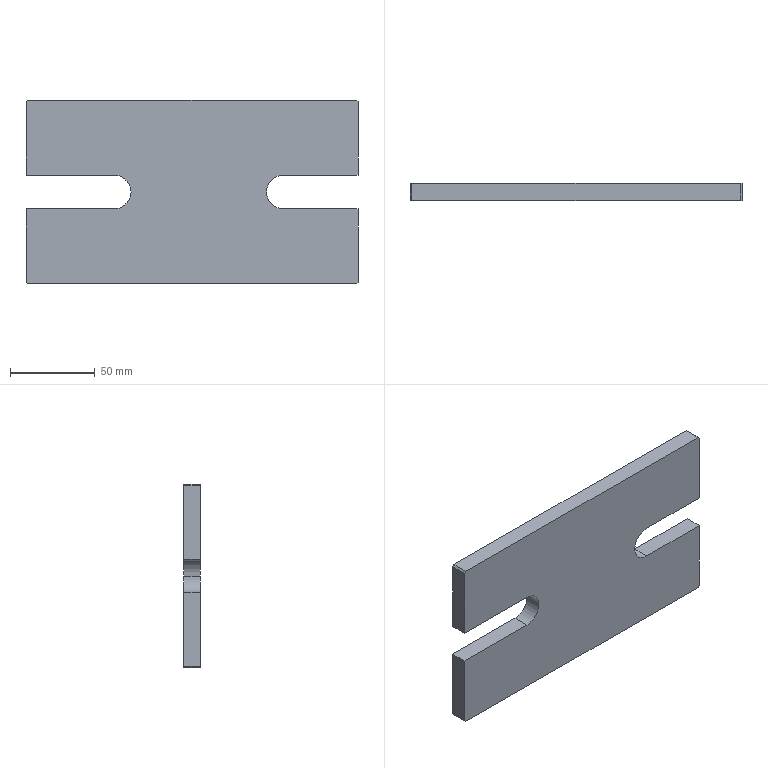Component | SolidWorks | 4GuidePlateAdjustmentPlate9.26-1 | 1 solid | 19 faces | box 196 x 10 x 108.5 mm | volume 190298 mm3 | plane 16 | cylinder 3 | commonest cylinder face diameters 20 x3 | material AISI 1045 Steel, Cold Drawn
build123d program:
from build123d import *

# Parameters (mm, degrees)
SKETCH1_W           = 160
SKETCH1_H           = 108.5
BOSS_EXTRUDE1_DEPTH = 10
CUT_EXTRUDE1_DEPTH  = 194.578
SKETCH3_W           = 10
SKETCH3_H           = 44.25
BOSS_EXTRUDE2_DEPTH = 14
SKETCH5_W           = 10
SKETCH5_H           = 44.25
BOSS_EXTRUDE3_DEPTH = 22
CHAMFER1_SIZE       = 1


with BuildPart() as part:
    # Sketch1 → Boss-Extrude1 (new body)
    with BuildSketch(Plane.XY):
        with Locations((80, -54.25)):
            Rectangle(SKETCH1_W, SKETCH1_H)
    extrude(amount=BOSS_EXTRUDE1_DEPTH)

    # Sketch2 → Cut-Extrude1 (cut, through all)
    with BuildSketch(Plane.XY.offset(10)):
        with BuildLine():
            Line((130, -44.25), (160, -44.25))
            Line((160, -44.25), (160, -64.25))
            Line((160, -64.25), (130, -64.25))
            ThreePointArc((130, -64.25), (120, -54.25), (130, -44.25))
        make_face()
        with BuildLine():
            Line((30, -44.25), (0, -44.25))
            Line((0, -44.25), (0, -64.25))
            Line((0, -64.25), (30, -64.25))
            ThreePointArc((30, -64.25), (40, -54.25), (30, -44.25))
        make_face()
    extrude(amount=-CUT_EXTRUDE1_DEPTH, mode=Mode.SUBTRACT)

    # Sketch3 → Boss-Extrude2 (add)
    with BuildSketch(Plane(origin=(160, 0, 0), x_dir=(0, 0, -1), z_dir=(1, 0, 0))):
        with Locations((-5, -86.375)):
            Rectangle(SKETCH3_W, SKETCH3_H)
        with Locations((-5, -22.125)):
            Rectangle(SKETCH3_W, SKETCH3_H)
    extrude(amount=BOSS_EXTRUDE2_DEPTH)

    # Sketch5 → Boss-Extrude3 (add)
    with BuildSketch(Plane.ZY):
        with Locations((5, -86.375)):
            Rectangle(SKETCH5_W, SKETCH5_H)
        with Locations((5, -22.125)):
            Rectangle(SKETCH5_W, SKETCH5_H)
    extrude(amount=BOSS_EXTRUDE3_DEPTH)

    # Chamfer1
    chamfer1_edges = [part.edges().sort_by_distance(p)[0] for p in [
        (174, -108.5, 5),
        (174, 0, 5),
        (-22, -108.5, 5),
        (-22, 0, 5),
    ]]
    chamfer(chamfer1_edges, length=CHAMFER1_SIZE)


solid = part.part

# Placed as in the assembly
solid = solid.moved(Location((112, -175, 69.5), (90, 0, 0)))